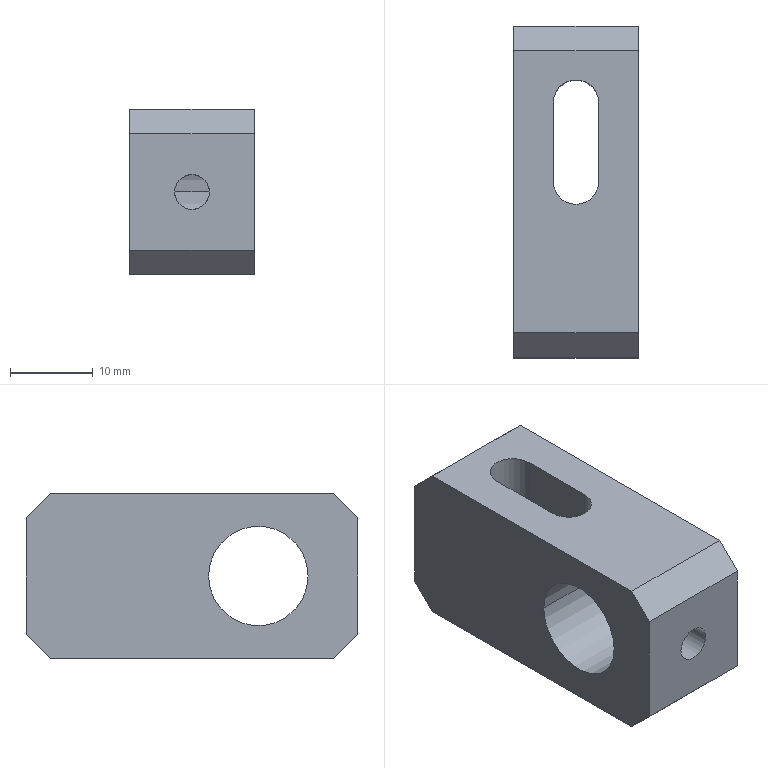Component | SolidWorks | 8TC-A15004-90-09A-1 | 1 solid | 19 faces | box 15 x 40 x 20 mm | volume 8429 mm3 | plane 12 | cylinder 7 | commonest cylinder face diameters 5.5 x3 4.2 x2 12 x2 | material A6061
STEP:
#1=CARTESIAN_POINT('',(-3.445,13.102,-3.346));
#2=VERTEX_POINT('',#1);
#3=CARTESIAN_POINT('',(-3.337,13.211,-3.346));
#4=VERTEX_POINT('',#3);
#5=CARTESIAN_POINT('',(-3.445,13.211,-3.346));
#6=DIRECTION('',(-0.,-0.,1.));
#7=DIRECTION('',(0.,-1.,0.));
#8=AXIS2_PLACEMENT_3D('',#5,#6,#7);
#9=CIRCLE('',#8,0.1083);
#10=EDGE_CURVE('',#2,#4,#9,.T.);
#11=ORIENTED_EDGE('',*,*,#10,.F.);
#12=CARTESIAN_POINT('',(-3.445,13.102,-2.559));
#13=VERTEX_POINT('',#12);
#14=CARTESIAN_POINT('',(-3.445,13.102,-2.559));
#15=DIRECTION('',(-0.,-0.,1.));
#16=VECTOR('',#15,39.37);
#17=LINE('',#14,#16);
#18=EDGE_CURVE('',#2,#13,#17,.T.);
#19=ORIENTED_EDGE('',*,*,#18,.T.);
#20=CARTESIAN_POINT('',(-3.337,13.211,-2.559));
#21=VERTEX_POINT('',#20);
#22=CARTESIAN_POINT('',(-3.445,13.211,-2.559));
#23=DIRECTION('',(-0.,-0.,1.));
#24=DIRECTION('',(0.,-1.,0.));
#25=AXIS2_PLACEMENT_3D('',#22,#23,#24);
#26=CIRCLE('',#25,0.1083);
#27=EDGE_CURVE('',#13,#21,#26,.T.);
#28=ORIENTED_EDGE('',*,*,#27,.T.);
#29=CARTESIAN_POINT('',(-3.337,13.211,-3.346));
#30=DIRECTION('',(-0.,0.,-1.));
#31=VECTOR('',#30,39.37);
#32=LINE('',#29,#31);
#33=EDGE_CURVE('',#21,#4,#32,.T.);
#34=ORIENTED_EDGE('',*,*,#33,.T.);
#35=EDGE_LOOP('',(#11,#19,#28,#34));
#36=FACE_OUTER_BOUND('',#35,.T.);
#37=CARTESIAN_POINT('',(-3.445,13.211,-2.559));
#38=DIRECTION('',(-0.,-0.,1.));
#39=DIRECTION('',(0.,-1.,0.));
#40=AXIS2_PLACEMENT_3D('',#37,#38,#39);
#41=CYLINDRICAL_SURFACE('',#40,0.1083);
#42=ADVANCED_FACE('',(#36),#41,.F.);
#43=CARTESIAN_POINT('',(-3.362,12.61,-2.953));
#44=VERTEX_POINT('',#43);
#45=CARTESIAN_POINT('',(-3.528,12.61,-2.953));
#46=VERTEX_POINT('',#45);
#47=CARTESIAN_POINT('',(-3.362,12.61,-2.953));
#48=CARTESIAN_POINT('',(-3.362,12.61,-2.958));
#49=CARTESIAN_POINT('',(-3.363,12.61,-2.964));
#50=CARTESIAN_POINT('',(-3.365,12.611,-2.974));
#51=CARTESIAN_POINT('',(-3.366,12.612,-2.98));
#52=CARTESIAN_POINT('',(-3.371,12.613,-2.99));
#53=CARTESIAN_POINT('',(-3.373,12.614,-2.994));
#54=CARTESIAN_POINT('',(-3.379,12.616,-3.003));
#55=CARTESIAN_POINT('',(-3.383,12.617,-3.007));
#56=CARTESIAN_POINT('',(-3.394,12.62,-3.019));
#57=CARTESIAN_POINT('',(-3.403,12.621,-3.025));
#58=CARTESIAN_POINT('',(-3.418,12.624,-3.031));
#59=CARTESIAN_POINT('',(-3.423,12.624,-3.033));
#60=CARTESIAN_POINT('',(-3.434,12.625,-3.035));
#61=CARTESIAN_POINT('',(-3.439,12.625,-3.035));
#62=CARTESIAN_POINT('',(-3.45,12.625,-3.035));
#63=CARTESIAN_POINT('',(-3.456,12.625,-3.035));
#64=CARTESIAN_POINT('',(-3.466,12.624,-3.033));
#65=CARTESIAN_POINT('',(-3.472,12.624,-3.031));
#66=CARTESIAN_POINT('',(-3.482,12.622,-3.027));
#67=CARTESIAN_POINT('',(-3.486,12.621,-3.024));
#68=CARTESIAN_POINT('',(-3.495,12.62,-3.018));
#69=CARTESIAN_POINT('',(-3.5,12.619,-3.015));
#70=CARTESIAN_POINT('',(-3.507,12.617,-3.007));
#71=CARTESIAN_POINT('',(-3.511,12.616,-3.003));
#72=CARTESIAN_POINT('',(-3.517,12.614,-2.994));
#73=CARTESIAN_POINT('',(-3.519,12.613,-2.989));
#74=CARTESIAN_POINT('',(-3.523,12.612,-2.98));
#75=CARTESIAN_POINT('',(-3.525,12.611,-2.974));
#76=CARTESIAN_POINT('',(-3.527,12.61,-2.964));
#77=CARTESIAN_POINT('',(-3.528,12.61,-2.958));
#78=CARTESIAN_POINT('',(-3.528,12.61,-2.953));
#79=B_SPLINE_CURVE_WITH_KNOTS('',3,(#47,#48,#49,#50,#51,#52,#53,#54,#55,#56,#57,#58,#59,#60,#61,#62,#63,#64,#65,#66,#67,#68,#69,#70,#71,#72,#73,#74,#75,#76,#77,#78),.UNSPECIFIED.,.F.,.F.,(4,2,2,2,2,2,2,2,2,2,2,2,2,2,2,4),(0.,0.0004136,0.0008273,0.001241,0.001655,0.002482,0.002896,0.003309,0.003723,0.004136,0.00455,0.004964,0.005377,0.005791,0.006205,0.006618),.UNSPECIFIED.);
#80=EDGE_CURVE('',#44,#46,#79,.T.);
#81=ORIENTED_EDGE('',*,*,#80,.T.);
#82=CARTESIAN_POINT('',(-3.528,12.374,-2.953));
#83=VERTEX_POINT('',#82);
#84=CARTESIAN_POINT('',(-3.528,12.374,-2.953));
#85=DIRECTION('',(-0.,-1.,-0.));
#86=VECTOR('',#85,39.37);
#87=LINE('',#84,#86);
#88=EDGE_CURVE('',#46,#83,#87,.T.);
#89=ORIENTED_EDGE('',*,*,#88,.T.);
#90=CARTESIAN_POINT('',(-3.362,12.374,-2.953));
#91=VERTEX_POINT('',#90);
#92=CARTESIAN_POINT('',(-3.445,12.374,-2.953));
#93=DIRECTION('',(-0.,-1.,-0.));
#94=DIRECTION('',(1.,0.,0.));
#95=AXIS2_PLACEMENT_3D('',#92,#93,#94);
#96=CIRCLE('',#95,0.08268);
#97=EDGE_CURVE('',#83,#91,#96,.T.);
#98=ORIENTED_EDGE('',*,*,#97,.T.);
#99=CARTESIAN_POINT('',(-3.362,12.374,-2.953));
#100=DIRECTION('',(-0.,-1.,-0.));
#101=VECTOR('',#100,39.37);
#102=LINE('',#99,#101);
#103=EDGE_CURVE('',#44,#91,#102,.T.);
#104=ORIENTED_EDGE('',*,*,#103,.F.);
#105=EDGE_LOOP('',(#81,#89,#98,#104));
#106=FACE_OUTER_BOUND('',#105,.T.);
#107=CARTESIAN_POINT('',(-3.445,12.374,-2.953));
#108=DIRECTION('',(-0.,-1.,-0.));
#109=DIRECTION('',(1.,0.,0.));
#110=AXIS2_PLACEMENT_3D('',#107,#108,#109);
#111=CYLINDRICAL_SURFACE('',#110,0.08268);
#112=ADVANCED_FACE('',(#106),#111,.F.);
#113=CARTESIAN_POINT('',(-3.74,13.083,-2.953));
#114=VERTEX_POINT('',#113);
#115=CARTESIAN_POINT('',(-3.74,12.61,-2.953));
#116=VERTEX_POINT('',#115);
#117=CARTESIAN_POINT('',(-3.74,12.846,-2.953));
#118=DIRECTION('',(-1.,0.,-0.));
#119=DIRECTION('',(0.,-1.,0.));
#120=AXIS2_PLACEMENT_3D('',#117,#118,#119);
#121=CIRCLE('',#120,0.2362);
#122=EDGE_CURVE('',#114,#116,#121,.T.);
#123=ORIENTED_EDGE('',*,*,#122,.T.);
#124=CARTESIAN_POINT('',(-3.74,12.61,-2.953));
#125=DIRECTION('',(1.,-0.,0.));
#126=VECTOR('',#125,39.37);
#127=LINE('',#124,#126);
#128=EDGE_CURVE('',#116,#46,#127,.T.);
#129=ORIENTED_EDGE('',*,*,#128,.T.);
#130=ORIENTED_EDGE('',*,*,#80,.F.);
#131=CARTESIAN_POINT('',(-3.15,12.61,-2.953));
#132=VERTEX_POINT('',#131);
#133=CARTESIAN_POINT('',(-3.74,12.61,-2.953));
#134=DIRECTION('',(1.,-0.,0.));
#135=VECTOR('',#134,39.37);
#136=LINE('',#133,#135);
#137=EDGE_CURVE('',#44,#132,#136,.T.);
#138=ORIENTED_EDGE('',*,*,#137,.T.);
#139=CARTESIAN_POINT('',(-3.15,13.083,-2.953));
#140=VERTEX_POINT('',#139);
#141=CARTESIAN_POINT('',(-3.15,12.846,-2.953));
#142=DIRECTION('',(-1.,0.,-0.));
#143=DIRECTION('',(0.,-1.,0.));
#144=AXIS2_PLACEMENT_3D('',#141,#142,#143);
#145=CIRCLE('',#144,0.2362);
#146=EDGE_CURVE('',#140,#132,#145,.T.);
#147=ORIENTED_EDGE('',*,*,#146,.F.);
#148=CARTESIAN_POINT('',(-3.74,13.083,-2.953));
#149=DIRECTION('',(1.,-0.,0.));
#150=VECTOR('',#149,39.37);
#151=LINE('',#148,#150);
#152=EDGE_CURVE('',#114,#140,#151,.T.);
#153=ORIENTED_EDGE('',*,*,#152,.F.);
#154=EDGE_LOOP('',(#123,#129,#130,#138,#147,#153));
#155=FACE_OUTER_BOUND('',#154,.T.);
#156=CARTESIAN_POINT('',(-3.74,12.846,-2.953));
#157=DIRECTION('',(1.,-0.,0.));
#158=DIRECTION('',(0.,1.,0.));
#159=AXIS2_PLACEMENT_3D('',#156,#157,#158);
#160=CYLINDRICAL_SURFACE('',#159,0.2362);
#161=ADVANCED_FACE('',(#155),#160,.F.);
#162=CARTESIAN_POINT('',(-3.15,12.492,-2.559));
#163=VERTEX_POINT('',#162);
#164=CARTESIAN_POINT('',(-3.15,13.831,-2.559));
#165=VERTEX_POINT('',#164);
#166=CARTESIAN_POINT('',(-3.15,12.374,-2.559));
#167=DIRECTION('',(0.,1.,0.));
#168=VECTOR('',#167,39.37);
#169=LINE('',#166,#168);
#170=EDGE_CURVE('',#163,#165,#169,.T.);
#171=ORIENTED_EDGE('',*,*,#170,.T.);
#172=CARTESIAN_POINT('',(-3.74,13.831,-2.559));
#173=VERTEX_POINT('',#172);
#174=CARTESIAN_POINT('',(-3.74,13.831,-2.559));
#175=DIRECTION('',(-1.,0.,-0.));
#176=VECTOR('',#175,39.37);
#177=LINE('',#174,#176);
#178=EDGE_CURVE('',#165,#173,#177,.T.);
#179=ORIENTED_EDGE('',*,*,#178,.T.);
#180=CARTESIAN_POINT('',(-3.74,12.492,-2.559));
#181=VERTEX_POINT('',#180);
#182=CARTESIAN_POINT('',(-3.74,12.374,-2.559));
#183=DIRECTION('',(-0.,-1.,-0.));
#184=VECTOR('',#183,39.37);
#185=LINE('',#182,#184);
#186=EDGE_CURVE('',#173,#181,#185,.T.);
#187=ORIENTED_EDGE('',*,*,#186,.T.);
#188=CARTESIAN_POINT('',(-3.15,12.492,-2.559));
#189=DIRECTION('',(1.,-0.,0.));
#190=VECTOR('',#189,39.37);
#191=LINE('',#188,#190);
#192=EDGE_CURVE('',#181,#163,#191,.T.);
#193=ORIENTED_EDGE('',*,*,#192,.T.);
#194=EDGE_LOOP('',(#171,#179,#187,#193));
#195=FACE_OUTER_BOUND('',#194,.T.);
#196=CARTESIAN_POINT('',(-3.337,13.585,-2.559));
#197=VERTEX_POINT('',#196);
#198=CARTESIAN_POINT('',(-3.553,13.585,-2.559));
#199=VERTEX_POINT('',#198);
#200=CARTESIAN_POINT('',(-3.445,13.585,-2.559));
#201=DIRECTION('',(-0.,-0.,1.));
#202=DIRECTION('',(0.,-1.,0.));
#203=AXIS2_PLACEMENT_3D('',#200,#201,#202);
#204=CIRCLE('',#203,0.1083);
#205=EDGE_CURVE('',#197,#199,#204,.T.);
#206=ORIENTED_EDGE('',*,*,#205,.F.);
#207=CARTESIAN_POINT('',(-3.337,13.585,-2.559));
#208=DIRECTION('',(-0.,-1.,-0.));
#209=VECTOR('',#208,39.37);
#210=LINE('',#207,#209);
#211=EDGE_CURVE('',#197,#21,#210,.T.);
#212=ORIENTED_EDGE('',*,*,#211,.T.);
#213=ORIENTED_EDGE('',*,*,#27,.F.);
#214=CARTESIAN_POINT('',(-3.553,13.211,-2.559));
#215=VERTEX_POINT('',#214);
#216=CARTESIAN_POINT('',(-3.445,13.211,-2.559));
#217=DIRECTION('',(-0.,-0.,1.));
#218=DIRECTION('',(0.,-1.,0.));
#219=AXIS2_PLACEMENT_3D('',#216,#217,#218);
#220=CIRCLE('',#219,0.1083);
#221=EDGE_CURVE('',#215,#13,#220,.T.);
#222=ORIENTED_EDGE('',*,*,#221,.F.);
#223=CARTESIAN_POINT('',(-3.553,13.585,-2.559));
#224=DIRECTION('',(-0.,-1.,-0.));
#225=VECTOR('',#224,39.37);
#226=LINE('',#223,#225);
#227=EDGE_CURVE('',#199,#215,#226,.T.);
#228=ORIENTED_EDGE('',*,*,#227,.F.);
#229=EDGE_LOOP('',(#206,#212,#213,#222,#228));
#230=FACE_BOUND('',#229,.T.);
#231=CARTESIAN_POINT('',(-3.445,13.161,-2.559));
#232=DIRECTION('',(-0.,-0.,1.));
#233=DIRECTION('',(-0.,-1.,-0.));
#234=AXIS2_PLACEMENT_3D('',#231,#232,#233);
#235=PLANE('',#234);
#236=ADVANCED_FACE('',(#195,#230),#235,.T.);
#237=CARTESIAN_POINT('',(-3.74,13.949,-2.677));
#238=VERTEX_POINT('',#237);
#239=CARTESIAN_POINT('',(-3.74,13.949,-3.228));
#240=VERTEX_POINT('',#239);
#241=CARTESIAN_POINT('',(-3.74,13.949,-2.559));
#242=DIRECTION('',(0.,0.,-1.));
#243=VECTOR('',#242,39.37);
#244=LINE('',#241,#243);
#245=EDGE_CURVE('',#238,#240,#244,.T.);
#246=ORIENTED_EDGE('',*,*,#245,.F.);
#247=CARTESIAN_POINT('',(-3.15,13.949,-2.677));
#248=VERTEX_POINT('',#247);
#249=CARTESIAN_POINT('',(-3.15,13.949,-2.677));
#250=DIRECTION('',(1.,-0.,0.));
#251=VECTOR('',#250,39.37);
#252=LINE('',#249,#251);
#253=EDGE_CURVE('',#238,#248,#252,.T.);
#254=ORIENTED_EDGE('',*,*,#253,.T.);
#255=CARTESIAN_POINT('',(-3.15,13.949,-3.228));
#256=VERTEX_POINT('',#255);
#257=CARTESIAN_POINT('',(-3.15,13.949,-2.559));
#258=DIRECTION('',(0.,0.,-1.));
#259=VECTOR('',#258,39.37);
#260=LINE('',#257,#259);
#261=EDGE_CURVE('',#248,#256,#260,.T.);
#262=ORIENTED_EDGE('',*,*,#261,.T.);
#263=CARTESIAN_POINT('',(-3.74,13.949,-3.228));
#264=DIRECTION('',(-1.,0.,-0.));
#265=VECTOR('',#264,39.37);
#266=LINE('',#263,#265);
#267=EDGE_CURVE('',#256,#240,#266,.T.);
#268=ORIENTED_EDGE('',*,*,#267,.T.);
#269=EDGE_LOOP('',(#246,#254,#262,#268));
#270=FACE_OUTER_BOUND('',#269,.T.);
#271=CARTESIAN_POINT('',(-3.74,13.949,-2.559));
#272=DIRECTION('',(-0.,-1.,-0.));
#273=DIRECTION('',(1.,-0.,0.));
#274=AXIS2_PLACEMENT_3D('',#271,#272,#273);
#275=PLANE('',#274);
#276=ADVANCED_FACE('',(#270),#275,.F.);
#277=ORIENTED_EDGE('',*,*,#122,.F.);
#278=CARTESIAN_POINT('',(-3.74,12.846,-2.953));
#279=DIRECTION('',(-1.,0.,-0.));
#280=DIRECTION('',(0.,-1.,0.));
#281=AXIS2_PLACEMENT_3D('',#278,#279,#280);
#282=CIRCLE('',#281,0.2362);
#283=EDGE_CURVE('',#116,#114,#282,.T.);
#284=ORIENTED_EDGE('',*,*,#283,.F.);
#285=EDGE_LOOP('',(#277,#284));
#286=FACE_BOUND('',#285,.T.);
#287=ORIENTED_EDGE('',*,*,#186,.F.);
#288=CARTESIAN_POINT('',(-3.74,13.831,-2.559));
#289=DIRECTION('',(0.,0.7071,-0.7071));
#290=VECTOR('',#289,39.37);
#291=LINE('',#288,#290);
#292=EDGE_CURVE('',#173,#238,#291,.T.);
#293=ORIENTED_EDGE('',*,*,#292,.T.);
#294=ORIENTED_EDGE('',*,*,#245,.T.);
#295=CARTESIAN_POINT('',(-3.74,13.831,-3.346));
#296=VERTEX_POINT('',#295);
#297=CARTESIAN_POINT('',(-3.74,13.949,-3.228));
#298=DIRECTION('',(0.,-0.7071,-0.7071));
#299=VECTOR('',#298,39.37);
#300=LINE('',#297,#299);
#301=EDGE_CURVE('',#240,#296,#300,.T.);
#302=ORIENTED_EDGE('',*,*,#301,.T.);
#303=CARTESIAN_POINT('',(-3.74,12.492,-3.346));
#304=VERTEX_POINT('',#303);
#305=CARTESIAN_POINT('',(-3.74,12.374,-3.346));
#306=DIRECTION('',(-0.,-1.,-0.));
#307=VECTOR('',#306,39.37);
#308=LINE('',#305,#307);
#309=EDGE_CURVE('',#296,#304,#308,.T.);
#310=ORIENTED_EDGE('',*,*,#309,.T.);
#311=CARTESIAN_POINT('',(-3.74,12.374,-3.228));
#312=VERTEX_POINT('',#311);
#313=CARTESIAN_POINT('',(-3.74,12.374,-3.228));
#314=DIRECTION('',(-0.,-0.7071,0.7071));
#315=VECTOR('',#314,39.37);
#316=LINE('',#313,#315);
#317=EDGE_CURVE('',#304,#312,#316,.T.);
#318=ORIENTED_EDGE('',*,*,#317,.T.);
#319=CARTESIAN_POINT('',(-3.74,12.374,-2.677));
#320=VERTEX_POINT('',#319);
#321=CARTESIAN_POINT('',(-3.74,12.374,-2.559));
#322=DIRECTION('',(0.,0.,-1.));
#323=VECTOR('',#322,39.37);
#324=LINE('',#321,#323);
#325=EDGE_CURVE('',#320,#312,#324,.T.);
#326=ORIENTED_EDGE('',*,*,#325,.F.);
#327=CARTESIAN_POINT('',(-3.74,12.492,-2.559));
#328=DIRECTION('',(-0.,0.7071,0.7071));
#329=VECTOR('',#328,39.37);
#330=LINE('',#327,#329);
#331=EDGE_CURVE('',#320,#181,#330,.T.);
#332=ORIENTED_EDGE('',*,*,#331,.T.);
#333=EDGE_LOOP('',(#287,#293,#294,#302,#310,#318,#326,#332));
#334=FACE_OUTER_BOUND('',#333,.T.);
#335=CARTESIAN_POINT('',(-3.74,12.374,-2.559));
#336=DIRECTION('',(1.,-0.,0.));
#337=DIRECTION('',(0.,1.,0.));
#338=AXIS2_PLACEMENT_3D('',#335,#336,#337);
#339=PLANE('',#338);
#340=ADVANCED_FACE('',(#286,#334),#339,.F.);
#341=CARTESIAN_POINT('',(-3.445,12.374,-2.953));
#342=DIRECTION('',(-0.,-1.,-0.));
#343=DIRECTION('',(1.,0.,0.));
#344=AXIS2_PLACEMENT_3D('',#341,#342,#343);
#345=CIRCLE('',#344,0.08268);
#346=EDGE_CURVE('',#91,#83,#345,.T.);
#347=ORIENTED_EDGE('',*,*,#346,.F.);
#348=ORIENTED_EDGE('',*,*,#97,.F.);
#349=EDGE_LOOP('',(#347,#348));
#350=FACE_BOUND('',#349,.T.);
#351=ORIENTED_EDGE('',*,*,#325,.T.);
#352=CARTESIAN_POINT('',(-3.15,12.374,-3.228));
#353=VERTEX_POINT('',#352);
#354=CARTESIAN_POINT('',(-3.74,12.374,-3.228));
#355=DIRECTION('',(1.,-0.,0.));
#356=VECTOR('',#355,39.37);
#357=LINE('',#354,#356);
#358=EDGE_CURVE('',#312,#353,#357,.T.);
#359=ORIENTED_EDGE('',*,*,#358,.T.);
#360=CARTESIAN_POINT('',(-3.15,12.374,-2.677));
#361=VERTEX_POINT('',#360);
#362=CARTESIAN_POINT('',(-3.15,12.374,-2.559));
#363=DIRECTION('',(0.,0.,-1.));
#364=VECTOR('',#363,39.37);
#365=LINE('',#362,#364);
#366=EDGE_CURVE('',#361,#353,#365,.T.);
#367=ORIENTED_EDGE('',*,*,#366,.F.);
#368=CARTESIAN_POINT('',(-3.74,12.374,-2.677));
#369=DIRECTION('',(-1.,0.,-0.));
#370=VECTOR('',#369,39.37);
#371=LINE('',#368,#370);
#372=EDGE_CURVE('',#361,#320,#371,.T.);
#373=ORIENTED_EDGE('',*,*,#372,.T.);
#374=EDGE_LOOP('',(#351,#359,#367,#373));
#375=FACE_OUTER_BOUND('',#374,.T.);
#376=CARTESIAN_POINT('',(-3.74,12.374,-2.559));
#377=DIRECTION('',(0.,1.,0.));
#378=DIRECTION('',(-1.,0.,-0.));
#379=AXIS2_PLACEMENT_3D('',#376,#377,#378);
#380=PLANE('',#379);
#381=ADVANCED_FACE('',(#350,#375),#380,.F.);
#382=ORIENTED_EDGE('',*,*,#146,.T.);
#383=CARTESIAN_POINT('',(-3.15,12.846,-2.953));
#384=DIRECTION('',(-1.,0.,-0.));
#385=DIRECTION('',(0.,-1.,0.));
#386=AXIS2_PLACEMENT_3D('',#383,#384,#385);
#387=CIRCLE('',#386,0.2362);
#388=EDGE_CURVE('',#132,#140,#387,.T.);
#389=ORIENTED_EDGE('',*,*,#388,.T.);
#390=EDGE_LOOP('',(#382,#389));
#391=FACE_BOUND('',#390,.T.);
#392=ORIENTED_EDGE('',*,*,#261,.F.);
#393=CARTESIAN_POINT('',(-3.15,13.831,-2.559));
#394=DIRECTION('',(-0.,-0.7071,0.7071));
#395=VECTOR('',#394,39.37);
#396=LINE('',#393,#395);
#397=EDGE_CURVE('',#248,#165,#396,.T.);
#398=ORIENTED_EDGE('',*,*,#397,.T.);
#399=ORIENTED_EDGE('',*,*,#170,.F.);
#400=CARTESIAN_POINT('',(-3.15,12.492,-2.559));
#401=DIRECTION('',(0.,-0.7071,-0.7071));
#402=VECTOR('',#401,39.37);
#403=LINE('',#400,#402);
#404=EDGE_CURVE('',#163,#361,#403,.T.);
#405=ORIENTED_EDGE('',*,*,#404,.T.);
#406=ORIENTED_EDGE('',*,*,#366,.T.);
#407=CARTESIAN_POINT('',(-3.15,12.492,-3.346));
#408=VERTEX_POINT('',#407);
#409=CARTESIAN_POINT('',(-3.15,12.374,-3.228));
#410=DIRECTION('',(0.,0.7071,-0.7071));
#411=VECTOR('',#410,39.37);
#412=LINE('',#409,#411);
#413=EDGE_CURVE('',#353,#408,#412,.T.);
#414=ORIENTED_EDGE('',*,*,#413,.T.);
#415=CARTESIAN_POINT('',(-3.15,13.831,-3.346));
#416=VERTEX_POINT('',#415);
#417=CARTESIAN_POINT('',(-3.15,12.374,-3.346));
#418=DIRECTION('',(0.,1.,0.));
#419=VECTOR('',#418,39.37);
#420=LINE('',#417,#419);
#421=EDGE_CURVE('',#408,#416,#420,.T.);
#422=ORIENTED_EDGE('',*,*,#421,.T.);
#423=CARTESIAN_POINT('',(-3.15,13.949,-3.228));
#424=DIRECTION('',(-0.,0.7071,0.7071));
#425=VECTOR('',#424,39.37);
#426=LINE('',#423,#425);
#427=EDGE_CURVE('',#416,#256,#426,.T.);
#428=ORIENTED_EDGE('',*,*,#427,.T.);
#429=EDGE_LOOP('',(#392,#398,#399,#405,#406,#414,#422,#428));
#430=FACE_OUTER_BOUND('',#429,.T.);
#431=CARTESIAN_POINT('',(-3.15,12.374,-2.559));
#432=DIRECTION('',(-1.,0.,-0.));
#433=DIRECTION('',(-0.,-1.,-0.));
#434=AXIS2_PLACEMENT_3D('',#431,#432,#433);
#435=PLANE('',#434);
#436=ADVANCED_FACE('',(#391,#430),#435,.F.);
#437=CARTESIAN_POINT('',(-3.337,13.585,-3.346));
#438=VERTEX_POINT('',#437);
#439=CARTESIAN_POINT('',(-3.553,13.585,-3.346));
#440=VERTEX_POINT('',#439);
#441=CARTESIAN_POINT('',(-3.445,13.585,-3.346));
#442=DIRECTION('',(-0.,-0.,1.));
#443=DIRECTION('',(0.,-1.,0.));
#444=AXIS2_PLACEMENT_3D('',#441,#442,#443);
#445=CIRCLE('',#444,0.1083);
#446=EDGE_CURVE('',#438,#440,#445,.T.);
#447=ORIENTED_EDGE('',*,*,#446,.T.);
#448=CARTESIAN_POINT('',(-3.553,13.211,-3.346));
#449=VERTEX_POINT('',#448);
#450=CARTESIAN_POINT('',(-3.553,13.585,-3.346));
#451=DIRECTION('',(-0.,-1.,-0.));
#452=VECTOR('',#451,39.37);
#453=LINE('',#450,#452);
#454=EDGE_CURVE('',#440,#449,#453,.T.);
#455=ORIENTED_EDGE('',*,*,#454,.T.);
#456=CARTESIAN_POINT('',(-3.445,13.211,-3.346));
#457=DIRECTION('',(-0.,-0.,1.));
#458=DIRECTION('',(0.,-1.,0.));
#459=AXIS2_PLACEMENT_3D('',#456,#457,#458);
#460=CIRCLE('',#459,0.1083);
#461=EDGE_CURVE('',#449,#2,#460,.T.);
#462=ORIENTED_EDGE('',*,*,#461,.T.);
#463=ORIENTED_EDGE('',*,*,#10,.T.);
#464=CARTESIAN_POINT('',(-3.337,13.585,-3.346));
#465=DIRECTION('',(-0.,-1.,-0.));
#466=VECTOR('',#465,39.37);
#467=LINE('',#464,#466);
#468=EDGE_CURVE('',#438,#4,#467,.T.);
#469=ORIENTED_EDGE('',*,*,#468,.F.);
#470=EDGE_LOOP('',(#447,#455,#462,#463,#469));
#471=FACE_BOUND('',#470,.T.);
#472=ORIENTED_EDGE('',*,*,#309,.F.);
#473=CARTESIAN_POINT('',(-3.445,13.831,-3.346));
#474=DIRECTION('',(1.,-0.,0.));
#475=VECTOR('',#474,39.37);
#476=LINE('',#473,#475);
#477=EDGE_CURVE('',#296,#416,#476,.T.);
#478=ORIENTED_EDGE('',*,*,#477,.T.);
#479=ORIENTED_EDGE('',*,*,#421,.F.);
#480=CARTESIAN_POINT('',(-3.445,12.492,-3.346));
#481=DIRECTION('',(-1.,0.,-0.));
#482=VECTOR('',#481,39.37);
#483=LINE('',#480,#482);
#484=EDGE_CURVE('',#408,#304,#483,.T.);
#485=ORIENTED_EDGE('',*,*,#484,.T.);
#486=EDGE_LOOP('',(#472,#478,#479,#485));
#487=FACE_OUTER_BOUND('',#486,.T.);
#488=CARTESIAN_POINT('',(-3.445,13.161,-3.346));
#489=DIRECTION('',(-0.,-0.,1.));
#490=DIRECTION('',(-0.,-1.,-0.));
#491=AXIS2_PLACEMENT_3D('',#488,#489,#490);
#492=PLANE('',#491);
#493=ADVANCED_FACE('',(#471,#487),#492,.F.);
#494=ORIENTED_EDGE('',*,*,#128,.F.);
#495=ORIENTED_EDGE('',*,*,#283,.T.);
#496=ORIENTED_EDGE('',*,*,#152,.T.);
#497=ORIENTED_EDGE('',*,*,#388,.F.);
#498=ORIENTED_EDGE('',*,*,#137,.F.);
#499=CARTESIAN_POINT('',(-3.528,12.61,-2.953));
#500=CARTESIAN_POINT('',(-3.528,12.61,-2.947));
#501=CARTESIAN_POINT('',(-3.527,12.61,-2.942));
#502=CARTESIAN_POINT('',(-3.525,12.611,-2.931));
#503=CARTESIAN_POINT('',(-3.523,12.612,-2.926));
#504=CARTESIAN_POINT('',(-3.519,12.613,-2.916));
#505=CARTESIAN_POINT('',(-3.517,12.614,-2.911));
#506=CARTESIAN_POINT('',(-3.511,12.616,-2.902));
#507=CARTESIAN_POINT('',(-3.507,12.617,-2.898));
#508=CARTESIAN_POINT('',(-3.496,12.62,-2.887));
#509=CARTESIAN_POINT('',(-3.487,12.621,-2.881));
#510=CARTESIAN_POINT('',(-3.472,12.624,-2.874));
#511=CARTESIAN_POINT('',(-3.466,12.624,-2.873));
#512=CARTESIAN_POINT('',(-3.456,12.625,-2.871));
#513=CARTESIAN_POINT('',(-3.45,12.625,-2.87));
#514=CARTESIAN_POINT('',(-3.439,12.625,-2.87));
#515=CARTESIAN_POINT('',(-3.434,12.625,-2.871));
#516=CARTESIAN_POINT('',(-3.423,12.624,-2.873));
#517=CARTESIAN_POINT('',(-3.418,12.624,-2.874));
#518=CARTESIAN_POINT('',(-3.403,12.621,-2.881));
#519=CARTESIAN_POINT('',(-3.394,12.62,-2.887));
#520=CARTESIAN_POINT('',(-3.383,12.617,-2.898));
#521=CARTESIAN_POINT('',(-3.379,12.616,-2.902));
#522=CARTESIAN_POINT('',(-3.373,12.614,-2.911));
#523=CARTESIAN_POINT('',(-3.371,12.613,-2.916));
#524=CARTESIAN_POINT('',(-3.366,12.612,-2.926));
#525=CARTESIAN_POINT('',(-3.365,12.611,-2.931));
#526=CARTESIAN_POINT('',(-3.363,12.61,-2.942));
#527=CARTESIAN_POINT('',(-3.362,12.61,-2.947));
#528=CARTESIAN_POINT('',(-3.362,12.61,-2.953));
#529=B_SPLINE_CURVE_WITH_KNOTS('',3,(#499,#500,#501,#502,#503,#504,#505,#506,#507,#508,#509,#510,#511,#512,#513,#514,#515,#516,#517,#518,#519,#520,#521,#522,#523,#524,#525,#526,#527,#528),.UNSPECIFIED.,.F.,.F.,(4,2,2,2,2,2,2,2,2,2,2,2,2,2,4),(0.006618,0.007032,0.007445,0.007859,0.008273,0.0091,0.009513,0.009927,0.01034,0.01075,0.01158,0.01199,0.01241,0.01282,0.01324),.UNSPECIFIED.);
#530=EDGE_CURVE('',#46,#44,#529,.T.);
#531=ORIENTED_EDGE('',*,*,#530,.F.);
#532=EDGE_LOOP('',(#494,#495,#496,#497,#498,#531));
#533=FACE_OUTER_BOUND('',#532,.T.);
#534=CARTESIAN_POINT('',(-3.74,12.846,-2.953));
#535=DIRECTION('',(1.,-0.,0.));
#536=DIRECTION('',(0.,1.,0.));
#537=AXIS2_PLACEMENT_3D('',#534,#535,#536);
#538=CYLINDRICAL_SURFACE('',#537,0.2362);
#539=ADVANCED_FACE('',(#533),#538,.F.);
#540=ORIENTED_EDGE('',*,*,#397,.F.);
#541=ORIENTED_EDGE('',*,*,#253,.F.);
#542=ORIENTED_EDGE('',*,*,#292,.F.);
#543=ORIENTED_EDGE('',*,*,#178,.F.);
#544=EDGE_LOOP('',(#540,#541,#542,#543));
#545=FACE_OUTER_BOUND('',#544,.T.);
#546=CARTESIAN_POINT('',(-3.445,13.831,-2.559));
#547=DIRECTION('',(-0.,0.7071,0.7071));
#548=DIRECTION('',(1.,-0.,0.));
#549=AXIS2_PLACEMENT_3D('',#546,#547,#548);
#550=PLANE('',#549);
#551=ADVANCED_FACE('',(#545),#550,.T.);
#552=ORIENTED_EDGE('',*,*,#427,.F.);
#553=ORIENTED_EDGE('',*,*,#477,.F.);
#554=ORIENTED_EDGE('',*,*,#301,.F.);
#555=ORIENTED_EDGE('',*,*,#267,.F.);
#556=EDGE_LOOP('',(#552,#553,#554,#555));
#557=FACE_OUTER_BOUND('',#556,.T.);
#558=CARTESIAN_POINT('',(-3.74,13.949,-3.228));
#559=DIRECTION('',(-0.,-0.7071,0.7071));
#560=DIRECTION('',(-1.,0.,-0.));
#561=AXIS2_PLACEMENT_3D('',#558,#559,#560);
#562=PLANE('',#561);
#563=ADVANCED_FACE('',(#557),#562,.F.);
#564=ORIENTED_EDGE('',*,*,#317,.F.);
#565=ORIENTED_EDGE('',*,*,#484,.F.);
#566=ORIENTED_EDGE('',*,*,#413,.F.);
#567=ORIENTED_EDGE('',*,*,#358,.F.);
#568=EDGE_LOOP('',(#564,#565,#566,#567));
#569=FACE_OUTER_BOUND('',#568,.T.);
#570=CARTESIAN_POINT('',(-3.74,12.374,-3.228));
#571=DIRECTION('',(-0.,0.7071,0.7071));
#572=DIRECTION('',(1.,-0.,0.));
#573=AXIS2_PLACEMENT_3D('',#570,#571,#572);
#574=PLANE('',#573);
#575=ADVANCED_FACE('',(#569),#574,.F.);
#576=ORIENTED_EDGE('',*,*,#331,.F.);
#577=ORIENTED_EDGE('',*,*,#372,.F.);
#578=ORIENTED_EDGE('',*,*,#404,.F.);
#579=ORIENTED_EDGE('',*,*,#192,.F.);
#580=EDGE_LOOP('',(#576,#577,#578,#579));
#581=FACE_OUTER_BOUND('',#580,.T.);
#582=CARTESIAN_POINT('',(-3.445,12.492,-2.559));
#583=DIRECTION('',(-0.,-0.7071,0.7071));
#584=DIRECTION('',(-1.,0.,-0.));
#585=AXIS2_PLACEMENT_3D('',#582,#583,#584);
#586=PLANE('',#585);
#587=ADVANCED_FACE('',(#581),#586,.T.);
#588=ORIENTED_EDGE('',*,*,#88,.F.);
#589=ORIENTED_EDGE('',*,*,#530,.T.);
#590=ORIENTED_EDGE('',*,*,#103,.T.);
#591=ORIENTED_EDGE('',*,*,#346,.T.);
#592=EDGE_LOOP('',(#588,#589,#590,#591));
#593=FACE_OUTER_BOUND('',#592,.T.);
#594=CARTESIAN_POINT('',(-3.445,12.374,-2.953));
#595=DIRECTION('',(-0.,-1.,-0.));
#596=DIRECTION('',(1.,0.,0.));
#597=AXIS2_PLACEMENT_3D('',#594,#595,#596);
#598=CYLINDRICAL_SURFACE('',#597,0.08268);
#599=ADVANCED_FACE('',(#593),#598,.F.);
#600=ORIENTED_EDGE('',*,*,#18,.F.);
#601=ORIENTED_EDGE('',*,*,#461,.F.);
#602=CARTESIAN_POINT('',(-3.553,13.211,-2.559));
#603=DIRECTION('',(0.,0.,-1.));
#604=VECTOR('',#603,39.37);
#605=LINE('',#602,#604);
#606=EDGE_CURVE('',#215,#449,#605,.T.);
#607=ORIENTED_EDGE('',*,*,#606,.F.);
#608=ORIENTED_EDGE('',*,*,#221,.T.);
#609=EDGE_LOOP('',(#600,#601,#607,#608));
#610=FACE_OUTER_BOUND('',#609,.T.);
#611=CARTESIAN_POINT('',(-3.445,13.211,-2.559));
#612=DIRECTION('',(-0.,-0.,1.));
#613=DIRECTION('',(0.,-1.,0.));
#614=AXIS2_PLACEMENT_3D('',#611,#612,#613);
#615=CYLINDRICAL_SURFACE('',#614,0.1083);
#616=ADVANCED_FACE('',(#610),#615,.F.);
#617=ORIENTED_EDGE('',*,*,#446,.F.);
#618=CARTESIAN_POINT('',(-3.337,13.585,-3.346));
#619=DIRECTION('',(-0.,0.,-1.));
#620=VECTOR('',#619,39.37);
#621=LINE('',#618,#620);
#622=EDGE_CURVE('',#197,#438,#621,.T.);
#623=ORIENTED_EDGE('',*,*,#622,.F.);
#624=ORIENTED_EDGE('',*,*,#205,.T.);
#625=CARTESIAN_POINT('',(-3.553,13.585,-2.559));
#626=DIRECTION('',(-0.,-0.,1.));
#627=VECTOR('',#626,39.37);
#628=LINE('',#625,#627);
#629=EDGE_CURVE('',#440,#199,#628,.T.);
#630=ORIENTED_EDGE('',*,*,#629,.F.);
#631=EDGE_LOOP('',(#617,#623,#624,#630));
#632=FACE_OUTER_BOUND('',#631,.T.);
#633=CARTESIAN_POINT('',(-3.445,13.585,-2.559));
#634=DIRECTION('',(-0.,-0.,1.));
#635=DIRECTION('',(0.,-1.,0.));
#636=AXIS2_PLACEMENT_3D('',#633,#634,#635);
#637=CYLINDRICAL_SURFACE('',#636,0.1083);
#638=ADVANCED_FACE('',(#632),#637,.F.);
#639=ORIENTED_EDGE('',*,*,#33,.F.);
#640=ORIENTED_EDGE('',*,*,#211,.F.);
#641=ORIENTED_EDGE('',*,*,#622,.T.);
#642=ORIENTED_EDGE('',*,*,#468,.T.);
#643=EDGE_LOOP('',(#639,#640,#641,#642));
#644=FACE_OUTER_BOUND('',#643,.T.);
#645=CARTESIAN_POINT('',(-3.337,13.585,-3.346));
#646=DIRECTION('',(-1.,0.,0.));
#647=DIRECTION('',(-0.,-1.,-0.));
#648=AXIS2_PLACEMENT_3D('',#645,#646,#647);
#649=PLANE('',#648);
#650=ADVANCED_FACE('',(#644),#649,.T.);
#651=ORIENTED_EDGE('',*,*,#606,.T.);
#652=ORIENTED_EDGE('',*,*,#454,.F.);
#653=ORIENTED_EDGE('',*,*,#629,.T.);
#654=ORIENTED_EDGE('',*,*,#227,.T.);
#655=EDGE_LOOP('',(#651,#652,#653,#654));
#656=FACE_OUTER_BOUND('',#655,.T.);
#657=CARTESIAN_POINT('',(-3.553,13.585,-2.559));
#658=DIRECTION('',(-1.,0.,-0.));
#659=DIRECTION('',(-0.,-1.,-0.));
#660=AXIS2_PLACEMENT_3D('',#657,#658,#659);
#661=PLANE('',#660);
#662=ADVANCED_FACE('',(#656),#661,.F.);
#663=CLOSED_SHELL('',(#42,#112,#161,#236,#276,#340,#381,#436,#493,#539,#551,#563,#575,#587,#599,#616,#638,#650,#662));
#664=MANIFOLD_SOLID_BREP('',#663);
#665=CARTESIAN_POINT('',(0.,0.,0.));
#666=DIRECTION('',(0.,0.,1.));
#667=DIRECTION('',(1.,0.,0.));
#668=AXIS2_PLACEMENT_3D('',#665,#666,#667);
#669=(LENGTH_UNIT()NAMED_UNIT(*)SI_UNIT($,.METRE.));
#670=LENGTH_MEASURE_WITH_UNIT(LENGTH_MEASURE(0.0254),#669);
#671=DIMENSIONAL_EXPONENTS(1.,0.,0.,0.,0.,0.,0.);
#672=(CONVERSION_BASED_UNIT('',#670)LENGTH_UNIT()NAMED_UNIT(#671));
#673=UNCERTAINTY_MEASURE_WITH_UNIT(LENGTH_MEASURE(0.00001),#672,'','');
#674=(NAMED_UNIT(*)PLANE_ANGLE_UNIT()SI_UNIT($,.RADIAN.));
#675=(NAMED_UNIT(*)SI_UNIT($,.STERADIAN.)SOLID_ANGLE_UNIT());
#676=(GEOMETRIC_REPRESENTATION_CONTEXT(3)GLOBAL_UNCERTAINTY_ASSIGNED_CONTEXT((#673))GLOBAL_UNIT_ASSIGNED_CONTEXT((#672,#674,#675))REPRESENTATION_CONTEXT('',''));
#677=ADVANCED_BREP_SHAPE_REPRESENTATION('',(#664,#668),#676);
#678=COLOUR_RGB('',0.7922,0.8196,0.9333);
#679=FILL_AREA_STYLE_COLOUR('',#678);
#680=FILL_AREA_STYLE('',(#679));
#681=SURFACE_STYLE_FILL_AREA(#680);
#682=SURFACE_SIDE_STYLE('',(#681));
#683=SURFACE_STYLE_USAGE(.BOTH.,#682);
#684=PRESENTATION_STYLE_ASSIGNMENT((#683));
#685=STYLED_ITEM('',(#684),#664);
#686=(LENGTH_UNIT()NAMED_UNIT(*)SI_UNIT($,.METRE.));
#687=LENGTH_MEASURE_WITH_UNIT(LENGTH_MEASURE(0.0254),#686);
#688=DIMENSIONAL_EXPONENTS(1.,0.,0.,0.,0.,0.,0.);
#689=(CONVERSION_BASED_UNIT('',#687)LENGTH_UNIT()NAMED_UNIT(#688));
#690=UNCERTAINTY_MEASURE_WITH_UNIT(LENGTH_MEASURE(0.00001),#689,'','');
#691=(NAMED_UNIT(*)PLANE_ANGLE_UNIT()SI_UNIT($,.RADIAN.));
#692=(NAMED_UNIT(*)SI_UNIT($,.STERADIAN.)SOLID_ANGLE_UNIT());
#693=(GEOMETRIC_REPRESENTATION_CONTEXT(3)GLOBAL_UNCERTAINTY_ASSIGNED_CONTEXT((#690))GLOBAL_UNIT_ASSIGNED_CONTEXT((#689,#691,#692))REPRESENTATION_CONTEXT('',''));
#694=MECHANICAL_DESIGN_GEOMETRIC_PRESENTATION_REPRESENTATION('',(#685),#693);
#695=PRESENTATION_LAYER_ASSIGNMENT('','',(#685));